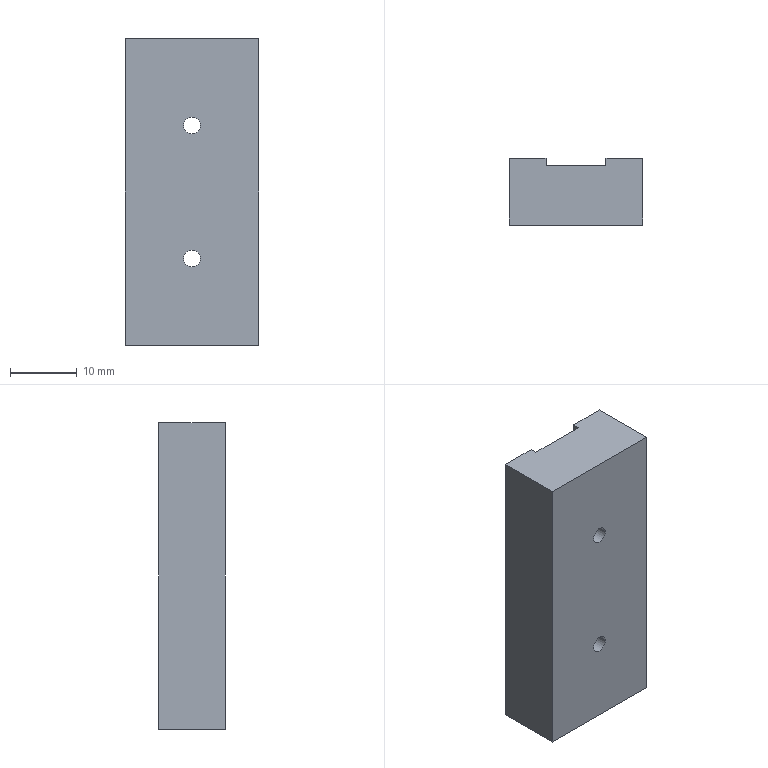Component | SolidWorks | P-SLJ-004-3_P-SLJ-004-002-1 | 1 solid | 22 faces | box 20 x 10 x 46 mm | volume 8495 mm3 | plane 10 | cylinder 8 | cone 4 | commonest cylinder face diameters 3.3 x4 2.5 x4 | material A3
build123d program:
from build123d import *

# Parameters (mm, degrees)
EXTRUDE1_DEPTH        = 23
M3_TAPPED_HOLE1_D     = 2.5
M4_TAPPED_HOLE2_D     = 3.3
M4_TAPPED_HOLE2_DEPTH = 11.5
M4_TAPPED_HOLE2_TIP   = 0.9914


with BuildPart() as part:
    # Sketch2 → Extrude1 (new, symmetric)
    with BuildSketch(Plane(origin=(0, 0, 0), x_dir=(0, 0, -1), z_dir=(1, 0, 0))):
        Polygon((4.5, 5), (10, 5), (10, -5), (-10, -5), (-10, 5), (-4.5, 5), (-4.5, 4), (4.5, 4), align=None)
    extrude(amount=EXTRUDE1_DEPTH, both=True)

    # M3 Tapped Hole1 (through all)
    with Locations(Plane(origin=(0, 4, 0), x_dir=(1, 0, 0), z_dir=(0, 1, 0))):
        with Locations((-10, 0), (10, 0)):
            Hole(M3_TAPPED_HOLE1_D / 2)

    # M4 Tapped Hole2
    with Locations(Plane.ZY.offset(23)):
        with Locations((5, 0), (-5, 0)):
            Hole(M4_TAPPED_HOLE2_D / 2, depth=M4_TAPPED_HOLE2_DEPTH)
            with Locations((0, 0, -(M4_TAPPED_HOLE2_DEPTH + M4_TAPPED_HOLE2_TIP / 2))):  # 118° drill point
                Cone(0, M4_TAPPED_HOLE2_D / 2, M4_TAPPED_HOLE2_TIP, mode=Mode.SUBTRACT)


solid = part.part

# Placed as in the assembly
solid = solid.moved(Location((-201.5, -45, 1287.634), (0, -90, 0)))
STEP:
#1=CARTESIAN_POINT('',(-8.065,-1.772,50.241));
#2=VERTEX_POINT('',#1);
#3=CARTESIAN_POINT('',(-8.195,-1.772,50.241));
#4=VERTEX_POINT('',#3);
#5=CARTESIAN_POINT('',(-8.13,-1.772,50.241));
#6=DIRECTION('',(-0.,0.,-1.));
#7=DIRECTION('',(-1.,0.,0.));
#8=AXIS2_PLACEMENT_3D('',#5,#6,#7);
#9=CIRCLE('',#8,0.06496);
#10=EDGE_CURVE('',#2,#4,#9,.T.);
#11=ORIENTED_EDGE('',*,*,#10,.F.);
#12=CARTESIAN_POINT('',(-8.065,-1.772,49.789));
#13=VERTEX_POINT('',#12);
#14=CARTESIAN_POINT('',(-8.065,-1.772,49.789));
#15=DIRECTION('',(-0.,0.,-1.));
#16=VECTOR('',#15,39.37);
#17=LINE('',#14,#16);
#18=EDGE_CURVE('',#2,#13,#17,.T.);
#19=ORIENTED_EDGE('',*,*,#18,.T.);
#20=CARTESIAN_POINT('',(-8.195,-1.772,49.789));
#21=VERTEX_POINT('',#20);
#22=CARTESIAN_POINT('',(-8.13,-1.772,49.789));
#23=DIRECTION('',(-0.,0.,-1.));
#24=DIRECTION('',(-1.,0.,0.));
#25=AXIS2_PLACEMENT_3D('',#22,#23,#24);
#26=CIRCLE('',#25,0.06496);
#27=EDGE_CURVE('',#13,#21,#26,.T.);
#28=ORIENTED_EDGE('',*,*,#27,.T.);
#29=CARTESIAN_POINT('',(-8.195,-1.772,49.789));
#30=DIRECTION('',(-0.,0.,-1.));
#31=VECTOR('',#30,39.37);
#32=LINE('',#29,#31);
#33=EDGE_CURVE('',#4,#21,#32,.T.);
#34=ORIENTED_EDGE('',*,*,#33,.F.);
#35=EDGE_LOOP('',(#11,#19,#28,#34));
#36=FACE_OUTER_BOUND('',#35,.T.);
#37=CARTESIAN_POINT('',(-8.13,-1.772,49.789));
#38=DIRECTION('',(-0.,0.,-1.));
#39=DIRECTION('',(-1.,0.,0.));
#40=AXIS2_PLACEMENT_3D('',#37,#38,#39);
#41=CYLINDRICAL_SURFACE('',#40,0.06496);
#42=ADVANCED_FACE('',(#36),#41,.F.);
#43=CARTESIAN_POINT('',(-8.13,-1.772,50.281));
#44=VERTEX_POINT('',#43);
#45=CARTESIAN_POINT('',(-8.195,-1.772,50.241));
#46=DIRECTION('',(-0.8572,0.,-0.515));
#47=VECTOR('',#46,39.37);
#48=LINE('',#45,#47);
#49=EDGE_CURVE('',#44,#4,#48,.T.);
#50=ORIENTED_EDGE('',*,*,#49,.F.);
#51=CARTESIAN_POINT('',(-8.065,-1.772,50.241));
#52=DIRECTION('',(0.8572,0.,-0.515));
#53=VECTOR('',#52,39.37);
#54=LINE('',#51,#53);
#55=EDGE_CURVE('',#44,#2,#54,.T.);
#56=ORIENTED_EDGE('',*,*,#55,.T.);
#57=ORIENTED_EDGE('',*,*,#10,.T.);
#58=EDGE_LOOP('',(#50,#56,#57));
#59=FACE_OUTER_BOUND('',#58,.T.);
#60=CARTESIAN_POINT('',(-8.13,-1.772,50.241));
#61=DIRECTION('',(-0.,0.,-1.));
#62=DIRECTION('',(-1.,0.,0.));
#63=AXIS2_PLACEMENT_3D('',#60,#61,#62);
#64=CONICAL_SURFACE('',#63,0.06496,1.03);
#65=ADVANCED_FACE('',(#59),#64,.F.);
#66=CARTESIAN_POINT('',(-7.671,-1.772,50.241));
#67=VERTEX_POINT('',#66);
#68=CARTESIAN_POINT('',(-7.801,-1.772,50.241));
#69=VERTEX_POINT('',#68);
#70=CARTESIAN_POINT('',(-7.736,-1.772,50.241));
#71=DIRECTION('',(-0.,0.,-1.));
#72=DIRECTION('',(-1.,0.,0.));
#73=AXIS2_PLACEMENT_3D('',#70,#71,#72);
#74=CIRCLE('',#73,0.06496);
#75=EDGE_CURVE('',#67,#69,#74,.T.);
#76=ORIENTED_EDGE('',*,*,#75,.F.);
#77=CARTESIAN_POINT('',(-7.671,-1.772,49.789));
#78=VERTEX_POINT('',#77);
#79=CARTESIAN_POINT('',(-7.671,-1.772,49.789));
#80=DIRECTION('',(-0.,0.,-1.));
#81=VECTOR('',#80,39.37);
#82=LINE('',#79,#81);
#83=EDGE_CURVE('',#67,#78,#82,.T.);
#84=ORIENTED_EDGE('',*,*,#83,.T.);
#85=CARTESIAN_POINT('',(-7.801,-1.772,49.789));
#86=VERTEX_POINT('',#85);
#87=CARTESIAN_POINT('',(-7.736,-1.772,49.789));
#88=DIRECTION('',(-0.,0.,-1.));
#89=DIRECTION('',(-1.,0.,0.));
#90=AXIS2_PLACEMENT_3D('',#87,#88,#89);
#91=CIRCLE('',#90,0.06496);
#92=EDGE_CURVE('',#78,#86,#91,.T.);
#93=ORIENTED_EDGE('',*,*,#92,.T.);
#94=CARTESIAN_POINT('',(-7.801,-1.772,49.789));
#95=DIRECTION('',(-0.,0.,-1.));
#96=VECTOR('',#95,39.37);
#97=LINE('',#94,#96);
#98=EDGE_CURVE('',#69,#86,#97,.T.);
#99=ORIENTED_EDGE('',*,*,#98,.F.);
#100=EDGE_LOOP('',(#76,#84,#93,#99));
#101=FACE_OUTER_BOUND('',#100,.T.);
#102=CARTESIAN_POINT('',(-7.736,-1.772,49.789));
#103=DIRECTION('',(-0.,0.,-1.));
#104=DIRECTION('',(-1.,0.,0.));
#105=AXIS2_PLACEMENT_3D('',#102,#103,#104);
#106=CYLINDRICAL_SURFACE('',#105,0.06496);
#107=ADVANCED_FACE('',(#101),#106,.F.);
#108=CARTESIAN_POINT('',(-7.736,-1.772,50.281));
#109=VERTEX_POINT('',#108);
#110=CARTESIAN_POINT('',(-7.801,-1.772,50.241));
#111=DIRECTION('',(-0.8572,0.,-0.515));
#112=VECTOR('',#111,39.37);
#113=LINE('',#110,#112);
#114=EDGE_CURVE('',#109,#69,#113,.T.);
#115=ORIENTED_EDGE('',*,*,#114,.F.);
#116=CARTESIAN_POINT('',(-7.671,-1.772,50.241));
#117=DIRECTION('',(0.8572,0.,-0.515));
#118=VECTOR('',#117,39.37);
#119=LINE('',#116,#118);
#120=EDGE_CURVE('',#109,#67,#119,.T.);
#121=ORIENTED_EDGE('',*,*,#120,.T.);
#122=ORIENTED_EDGE('',*,*,#75,.T.);
#123=EDGE_LOOP('',(#115,#121,#122));
#124=FACE_OUTER_BOUND('',#123,.T.);
#125=CARTESIAN_POINT('',(-7.736,-1.772,50.241));
#126=DIRECTION('',(-0.,0.,-1.));
#127=DIRECTION('',(-1.,0.,0.));
#128=AXIS2_PLACEMENT_3D('',#125,#126,#127);
#129=CONICAL_SURFACE('',#128,0.06496,1.03);
#130=ADVANCED_FACE('',(#124),#129,.F.);
#131=CARTESIAN_POINT('',(-7.884,-1.969,50.301));
#132=VERTEX_POINT('',#131);
#133=CARTESIAN_POINT('',(-7.982,-1.969,50.301));
#134=VERTEX_POINT('',#133);
#135=CARTESIAN_POINT('',(-7.933,-1.969,50.301));
#136=DIRECTION('',(0.,1.,0.));
#137=DIRECTION('',(-1.,0.,0.));
#138=AXIS2_PLACEMENT_3D('',#135,#136,#137);
#139=CIRCLE('',#138,0.04921);
#140=EDGE_CURVE('',#132,#134,#139,.T.);
#141=ORIENTED_EDGE('',*,*,#140,.F.);
#142=CARTESIAN_POINT('',(-7.884,-1.614,50.301));
#143=VERTEX_POINT('',#142);
#144=CARTESIAN_POINT('',(-7.884,-1.614,50.301));
#145=DIRECTION('',(0.,1.,0.));
#146=VECTOR('',#145,39.37);
#147=LINE('',#144,#146);
#148=EDGE_CURVE('',#132,#143,#147,.T.);
#149=ORIENTED_EDGE('',*,*,#148,.T.);
#150=CARTESIAN_POINT('',(-7.982,-1.614,50.301));
#151=VERTEX_POINT('',#150);
#152=CARTESIAN_POINT('',(-7.933,-1.614,50.301));
#153=DIRECTION('',(0.,1.,0.));
#154=DIRECTION('',(-1.,0.,0.));
#155=AXIS2_PLACEMENT_3D('',#152,#153,#154);
#156=CIRCLE('',#155,0.04921);
#157=EDGE_CURVE('',#143,#151,#156,.T.);
#158=ORIENTED_EDGE('',*,*,#157,.T.);
#159=CARTESIAN_POINT('',(-7.982,-1.614,50.301));
#160=DIRECTION('',(0.,1.,0.));
#161=VECTOR('',#160,39.37);
#162=LINE('',#159,#161);
#163=EDGE_CURVE('',#134,#151,#162,.T.);
#164=ORIENTED_EDGE('',*,*,#163,.F.);
#165=EDGE_LOOP('',(#141,#149,#158,#164));
#166=FACE_OUTER_BOUND('',#165,.T.);
#167=CARTESIAN_POINT('',(-7.933,-1.614,50.301));
#168=DIRECTION('',(0.,1.,0.));
#169=DIRECTION('',(-1.,0.,0.));
#170=AXIS2_PLACEMENT_3D('',#167,#168,#169);
#171=CYLINDRICAL_SURFACE('',#170,0.04921);
#172=ADVANCED_FACE('',(#166),#171,.F.);
#173=CARTESIAN_POINT('',(-7.884,-1.969,51.088));
#174=VERTEX_POINT('',#173);
#175=CARTESIAN_POINT('',(-7.982,-1.969,51.088));
#176=VERTEX_POINT('',#175);
#177=CARTESIAN_POINT('',(-7.933,-1.969,51.088));
#178=DIRECTION('',(0.,1.,0.));
#179=DIRECTION('',(-1.,0.,0.));
#180=AXIS2_PLACEMENT_3D('',#177,#178,#179);
#181=CIRCLE('',#180,0.04921);
#182=EDGE_CURVE('',#174,#176,#181,.T.);
#183=ORIENTED_EDGE('',*,*,#182,.F.);
#184=CARTESIAN_POINT('',(-7.884,-1.614,51.088));
#185=VERTEX_POINT('',#184);
#186=CARTESIAN_POINT('',(-7.884,-1.614,51.088));
#187=DIRECTION('',(0.,1.,0.));
#188=VECTOR('',#187,39.37);
#189=LINE('',#186,#188);
#190=EDGE_CURVE('',#174,#185,#189,.T.);
#191=ORIENTED_EDGE('',*,*,#190,.T.);
#192=CARTESIAN_POINT('',(-7.982,-1.614,51.088));
#193=VERTEX_POINT('',#192);
#194=CARTESIAN_POINT('',(-7.933,-1.614,51.088));
#195=DIRECTION('',(0.,1.,0.));
#196=DIRECTION('',(-1.,0.,0.));
#197=AXIS2_PLACEMENT_3D('',#194,#195,#196);
#198=CIRCLE('',#197,0.04921);
#199=EDGE_CURVE('',#185,#193,#198,.T.);
#200=ORIENTED_EDGE('',*,*,#199,.T.);
#201=CARTESIAN_POINT('',(-7.982,-1.614,51.088));
#202=DIRECTION('',(0.,1.,0.));
#203=VECTOR('',#202,39.37);
#204=LINE('',#201,#203);
#205=EDGE_CURVE('',#176,#193,#204,.T.);
#206=ORIENTED_EDGE('',*,*,#205,.F.);
#207=EDGE_LOOP('',(#183,#191,#200,#206));
#208=FACE_OUTER_BOUND('',#207,.T.);
#209=CARTESIAN_POINT('',(-7.933,-1.614,51.088));
#210=DIRECTION('',(0.,1.,0.));
#211=DIRECTION('',(-1.,0.,0.));
#212=AXIS2_PLACEMENT_3D('',#209,#210,#211);
#213=CYLINDRICAL_SURFACE('',#212,0.04921);
#214=ADVANCED_FACE('',(#208),#213,.F.);
#215=CARTESIAN_POINT('',(-7.539,-1.969,49.789));
#216=VERTEX_POINT('',#215);
#217=CARTESIAN_POINT('',(-7.539,-1.575,49.789));
#218=VERTEX_POINT('',#217);
#219=CARTESIAN_POINT('',(-7.539,-1.969,49.789));
#220=DIRECTION('',(-0.,1.,0.));
#221=VECTOR('',#220,39.37);
#222=LINE('',#219,#221);
#223=EDGE_CURVE('',#216,#218,#222,.T.);
#224=ORIENTED_EDGE('',*,*,#223,.T.);
#225=CARTESIAN_POINT('',(-7.539,-1.575,51.6));
#226=VERTEX_POINT('',#225);
#227=CARTESIAN_POINT('',(-7.539,-1.575,51.6));
#228=DIRECTION('',(-0.,0.,-1.));
#229=VECTOR('',#228,39.37);
#230=LINE('',#227,#229);
#231=EDGE_CURVE('',#226,#218,#230,.T.);
#232=ORIENTED_EDGE('',*,*,#231,.F.);
#233=CARTESIAN_POINT('',(-7.539,-1.969,51.6));
#234=VERTEX_POINT('',#233);
#235=CARTESIAN_POINT('',(-7.539,-1.969,51.6));
#236=DIRECTION('',(-0.,1.,0.));
#237=VECTOR('',#236,39.37);
#238=LINE('',#235,#237);
#239=EDGE_CURVE('',#234,#226,#238,.T.);
#240=ORIENTED_EDGE('',*,*,#239,.F.);
#241=CARTESIAN_POINT('',(-7.539,-1.969,51.6));
#242=DIRECTION('',(-0.,0.,-1.));
#243=VECTOR('',#242,39.37);
#244=LINE('',#241,#243);
#245=EDGE_CURVE('',#234,#216,#244,.T.);
#246=ORIENTED_EDGE('',*,*,#245,.T.);
#247=EDGE_LOOP('',(#224,#232,#240,#246));
#248=FACE_OUTER_BOUND('',#247,.T.);
#249=CARTESIAN_POINT('',(-7.539,-1.969,51.6));
#250=DIRECTION('',(-1.,-0.,0.));
#251=DIRECTION('',(0.,-1.,-0.));
#252=AXIS2_PLACEMENT_3D('',#249,#250,#251);
#253=PLANE('',#252);
#254=ADVANCED_FACE('',(#248),#253,.F.);
#255=CARTESIAN_POINT('',(-7.756,-1.575,49.789));
#256=VERTEX_POINT('',#255);
#257=CARTESIAN_POINT('',(-7.756,-1.575,49.789));
#258=DIRECTION('',(-1.,0.,0.));
#259=VECTOR('',#258,39.37);
#260=LINE('',#257,#259);
#261=EDGE_CURVE('',#218,#256,#260,.T.);
#262=ORIENTED_EDGE('',*,*,#261,.T.);
#263=CARTESIAN_POINT('',(-7.756,-1.575,51.6));
#264=VERTEX_POINT('',#263);
#265=CARTESIAN_POINT('',(-7.756,-1.575,51.6));
#266=DIRECTION('',(-0.,0.,-1.));
#267=VECTOR('',#266,39.37);
#268=LINE('',#265,#267);
#269=EDGE_CURVE('',#264,#256,#268,.T.);
#270=ORIENTED_EDGE('',*,*,#269,.F.);
#271=CARTESIAN_POINT('',(-7.756,-1.575,51.6));
#272=DIRECTION('',(-1.,0.,0.));
#273=VECTOR('',#272,39.37);
#274=LINE('',#271,#273);
#275=EDGE_CURVE('',#226,#264,#274,.T.);
#276=ORIENTED_EDGE('',*,*,#275,.F.);
#277=ORIENTED_EDGE('',*,*,#231,.T.);
#278=EDGE_LOOP('',(#262,#270,#276,#277));
#279=FACE_OUTER_BOUND('',#278,.T.);
#280=CARTESIAN_POINT('',(-7.756,-1.575,51.6));
#281=DIRECTION('',(-0.,-1.,-0.));
#282=DIRECTION('',(1.,-0.,-0.));
#283=AXIS2_PLACEMENT_3D('',#280,#281,#282);
#284=PLANE('',#283);
#285=ADVANCED_FACE('',(#279),#284,.F.);
#286=CARTESIAN_POINT('',(-7.756,-1.614,49.789));
#287=VERTEX_POINT('',#286);
#288=CARTESIAN_POINT('',(-7.756,-1.575,49.789));
#289=DIRECTION('',(-0.,-1.,-0.));
#290=VECTOR('',#289,39.37);
#291=LINE('',#288,#290);
#292=EDGE_CURVE('',#256,#287,#291,.T.);
#293=ORIENTED_EDGE('',*,*,#292,.T.);
#294=CARTESIAN_POINT('',(-7.756,-1.614,51.6));
#295=VERTEX_POINT('',#294);
#296=CARTESIAN_POINT('',(-7.756,-1.614,51.6));
#297=DIRECTION('',(-0.,0.,-1.));
#298=VECTOR('',#297,39.37);
#299=LINE('',#296,#298);
#300=EDGE_CURVE('',#295,#287,#299,.T.);
#301=ORIENTED_EDGE('',*,*,#300,.F.);
#302=CARTESIAN_POINT('',(-7.756,-1.575,51.6));
#303=DIRECTION('',(-0.,-1.,-0.));
#304=VECTOR('',#303,39.37);
#305=LINE('',#302,#304);
#306=EDGE_CURVE('',#264,#295,#305,.T.);
#307=ORIENTED_EDGE('',*,*,#306,.F.);
#308=ORIENTED_EDGE('',*,*,#269,.T.);
#309=EDGE_LOOP('',(#293,#301,#307,#308));
#310=FACE_OUTER_BOUND('',#309,.T.);
#311=CARTESIAN_POINT('',(-7.756,-1.575,51.6));
#312=DIRECTION('',(1.,-0.,-0.));
#313=DIRECTION('',(-0.,0.,-1.));
#314=AXIS2_PLACEMENT_3D('',#311,#312,#313);
#315=PLANE('',#314);
#316=ADVANCED_FACE('',(#310),#315,.F.);
#317=CARTESIAN_POINT('',(-7.933,-1.614,50.301));
#318=DIRECTION('',(0.,1.,0.));
#319=DIRECTION('',(-1.,0.,0.));
#320=AXIS2_PLACEMENT_3D('',#317,#318,#319);
#321=CIRCLE('',#320,0.04921);
#322=EDGE_CURVE('',#151,#143,#321,.T.);
#323=ORIENTED_EDGE('',*,*,#322,.F.);
#324=ORIENTED_EDGE('',*,*,#157,.F.);
#325=EDGE_LOOP('',(#323,#324));
#326=FACE_BOUND('',#325,.T.);
#327=CARTESIAN_POINT('',(-7.933,-1.614,51.088));
#328=DIRECTION('',(0.,1.,0.));
#329=DIRECTION('',(-1.,0.,0.));
#330=AXIS2_PLACEMENT_3D('',#327,#328,#329);
#331=CIRCLE('',#330,0.04921);
#332=EDGE_CURVE('',#193,#185,#331,.T.);
#333=ORIENTED_EDGE('',*,*,#332,.F.);
#334=ORIENTED_EDGE('',*,*,#199,.F.);
#335=EDGE_LOOP('',(#333,#334));
#336=FACE_BOUND('',#335,.T.);
#337=CARTESIAN_POINT('',(-8.11,-1.614,49.789));
#338=VERTEX_POINT('',#337);
#339=CARTESIAN_POINT('',(-8.11,-1.614,49.789));
#340=DIRECTION('',(-1.,0.,0.));
#341=VECTOR('',#340,39.37);
#342=LINE('',#339,#341);
#343=EDGE_CURVE('',#287,#338,#342,.T.);
#344=ORIENTED_EDGE('',*,*,#343,.T.);
#345=CARTESIAN_POINT('',(-8.11,-1.614,51.6));
#346=VERTEX_POINT('',#345);
#347=CARTESIAN_POINT('',(-8.11,-1.614,51.6));
#348=DIRECTION('',(-0.,0.,-1.));
#349=VECTOR('',#348,39.37);
#350=LINE('',#347,#349);
#351=EDGE_CURVE('',#346,#338,#350,.T.);
#352=ORIENTED_EDGE('',*,*,#351,.F.);
#353=CARTESIAN_POINT('',(-8.11,-1.614,51.6));
#354=DIRECTION('',(-1.,0.,0.));
#355=VECTOR('',#354,39.37);
#356=LINE('',#353,#355);
#357=EDGE_CURVE('',#295,#346,#356,.T.);
#358=ORIENTED_EDGE('',*,*,#357,.F.);
#359=ORIENTED_EDGE('',*,*,#300,.T.);
#360=EDGE_LOOP('',(#344,#352,#358,#359));
#361=FACE_OUTER_BOUND('',#360,.T.);
#362=CARTESIAN_POINT('',(-8.11,-1.614,51.6));
#363=DIRECTION('',(-0.,-1.,-0.));
#364=DIRECTION('',(1.,-0.,-0.));
#365=AXIS2_PLACEMENT_3D('',#362,#363,#364);
#366=PLANE('',#365);
#367=ADVANCED_FACE('',(#326,#336,#361),#366,.F.);
#368=CARTESIAN_POINT('',(-8.11,-1.575,49.789));
#369=VERTEX_POINT('',#368);
#370=CARTESIAN_POINT('',(-8.11,-1.575,49.789));
#371=DIRECTION('',(0.,1.,0.));
#372=VECTOR('',#371,39.37);
#373=LINE('',#370,#372);
#374=EDGE_CURVE('',#338,#369,#373,.T.);
#375=ORIENTED_EDGE('',*,*,#374,.T.);
#376=CARTESIAN_POINT('',(-8.11,-1.575,51.6));
#377=VERTEX_POINT('',#376);
#378=CARTESIAN_POINT('',(-8.11,-1.575,51.6));
#379=DIRECTION('',(-0.,0.,-1.));
#380=VECTOR('',#379,39.37);
#381=LINE('',#378,#380);
#382=EDGE_CURVE('',#377,#369,#381,.T.);
#383=ORIENTED_EDGE('',*,*,#382,.F.);
#384=CARTESIAN_POINT('',(-8.11,-1.575,51.6));
#385=DIRECTION('',(0.,1.,0.));
#386=VECTOR('',#385,39.37);
#387=LINE('',#384,#386);
#388=EDGE_CURVE('',#346,#377,#387,.T.);
#389=ORIENTED_EDGE('',*,*,#388,.F.);
#390=ORIENTED_EDGE('',*,*,#351,.T.);
#391=EDGE_LOOP('',(#375,#383,#389,#390));
#392=FACE_OUTER_BOUND('',#391,.T.);
#393=CARTESIAN_POINT('',(-8.11,-1.575,51.6));
#394=DIRECTION('',(-1.,0.,0.));
#395=DIRECTION('',(0.,-0.,1.));
#396=AXIS2_PLACEMENT_3D('',#393,#394,#395);
#397=PLANE('',#396);
#398=ADVANCED_FACE('',(#392),#397,.F.);
#399=CARTESIAN_POINT('',(-8.327,-1.575,49.789));
#400=VERTEX_POINT('',#399);
#401=CARTESIAN_POINT('',(-8.327,-1.575,49.789));
#402=DIRECTION('',(-1.,-0.,0.));
#403=VECTOR('',#402,39.37);
#404=LINE('',#401,#403);
#405=EDGE_CURVE('',#369,#400,#404,.T.);
#406=ORIENTED_EDGE('',*,*,#405,.T.);
#407=CARTESIAN_POINT('',(-8.327,-1.575,51.6));
#408=VERTEX_POINT('',#407);
#409=CARTESIAN_POINT('',(-8.327,-1.575,51.6));
#410=DIRECTION('',(-0.,0.,-1.));
#411=VECTOR('',#410,39.37);
#412=LINE('',#409,#411);
#413=EDGE_CURVE('',#408,#400,#412,.T.);
#414=ORIENTED_EDGE('',*,*,#413,.F.);
#415=CARTESIAN_POINT('',(-8.327,-1.575,51.6));
#416=DIRECTION('',(-1.,-0.,0.));
#417=VECTOR('',#416,39.37);
#418=LINE('',#415,#417);
#419=EDGE_CURVE('',#377,#408,#418,.T.);
#420=ORIENTED_EDGE('',*,*,#419,.F.);
#421=ORIENTED_EDGE('',*,*,#382,.T.);
#422=EDGE_LOOP('',(#406,#414,#420,#421));
#423=FACE_OUTER_BOUND('',#422,.T.);
#424=CARTESIAN_POINT('',(-8.327,-1.575,51.6));
#425=DIRECTION('',(0.,-1.,-0.));
#426=DIRECTION('',(1.,0.,-0.));
#427=AXIS2_PLACEMENT_3D('',#424,#425,#426);
#428=PLANE('',#427);
#429=ADVANCED_FACE('',(#423),#428,.F.);
#430=CARTESIAN_POINT('',(-8.327,-1.969,49.789));
#431=VERTEX_POINT('',#430);
#432=CARTESIAN_POINT('',(-8.327,-1.969,49.789));
#433=DIRECTION('',(-0.,-1.,-0.));
#434=VECTOR('',#433,39.37);
#435=LINE('',#432,#434);
#436=EDGE_CURVE('',#400,#431,#435,.T.);
#437=ORIENTED_EDGE('',*,*,#436,.T.);
#438=CARTESIAN_POINT('',(-8.327,-1.969,51.6));
#439=VERTEX_POINT('',#438);
#440=CARTESIAN_POINT('',(-8.327,-1.969,51.6));
#441=DIRECTION('',(-0.,0.,-1.));
#442=VECTOR('',#441,39.37);
#443=LINE('',#440,#442);
#444=EDGE_CURVE('',#439,#431,#443,.T.);
#445=ORIENTED_EDGE('',*,*,#444,.F.);
#446=CARTESIAN_POINT('',(-8.327,-1.969,51.6));
#447=DIRECTION('',(-0.,-1.,-0.));
#448=VECTOR('',#447,39.37);
#449=LINE('',#446,#448);
#450=EDGE_CURVE('',#408,#439,#449,.T.);
#451=ORIENTED_EDGE('',*,*,#450,.F.);
#452=ORIENTED_EDGE('',*,*,#413,.T.);
#453=EDGE_LOOP('',(#437,#445,#451,#452));
#454=FACE_OUTER_BOUND('',#453,.T.);
#455=CARTESIAN_POINT('',(-8.327,-1.969,51.6));
#456=DIRECTION('',(1.,-0.,-0.));
#457=DIRECTION('',(-0.,0.,-1.));
#458=AXIS2_PLACEMENT_3D('',#455,#456,#457);
#459=PLANE('',#458);
#460=ADVANCED_FACE('',(#454),#459,.F.);
#461=CARTESIAN_POINT('',(-7.933,-1.969,50.301));
#462=DIRECTION('',(0.,1.,0.));
#463=DIRECTION('',(-1.,0.,0.));
#464=AXIS2_PLACEMENT_3D('',#461,#462,#463);
#465=CIRCLE('',#464,0.04921);
#466=EDGE_CURVE('',#134,#132,#465,.T.);
#467=ORIENTED_EDGE('',*,*,#466,.T.);
#468=ORIENTED_EDGE('',*,*,#140,.T.);
#469=EDGE_LOOP('',(#467,#468));
#470=FACE_BOUND('',#469,.T.);
#471=CARTESIAN_POINT('',(-7.933,-1.969,51.088));
#472=DIRECTION('',(0.,1.,0.));
#473=DIRECTION('',(-1.,0.,0.));
#474=AXIS2_PLACEMENT_3D('',#471,#472,#473);
#475=CIRCLE('',#474,0.04921);
#476=EDGE_CURVE('',#176,#174,#475,.T.);
#477=ORIENTED_EDGE('',*,*,#476,.T.);
#478=ORIENTED_EDGE('',*,*,#182,.T.);
#479=EDGE_LOOP('',(#477,#478));
#480=FACE_BOUND('',#479,.T.);
#481=CARTESIAN_POINT('',(-8.327,-1.969,49.789));
#482=DIRECTION('',(1.,-0.,-0.));
#483=VECTOR('',#482,39.37);
#484=LINE('',#481,#483);
#485=EDGE_CURVE('',#431,#216,#484,.T.);
#486=ORIENTED_EDGE('',*,*,#485,.T.);
#487=ORIENTED_EDGE('',*,*,#245,.F.);
#488=CARTESIAN_POINT('',(-8.327,-1.969,51.6));
#489=DIRECTION('',(1.,-0.,-0.));
#490=VECTOR('',#489,39.37);
#491=LINE('',#488,#490);
#492=EDGE_CURVE('',#439,#234,#491,.T.);
#493=ORIENTED_EDGE('',*,*,#492,.F.);
#494=ORIENTED_EDGE('',*,*,#444,.T.);
#495=EDGE_LOOP('',(#486,#487,#493,#494));
#496=FACE_OUTER_BOUND('',#495,.T.);
#497=CARTESIAN_POINT('',(-8.327,-1.969,51.6));
#498=DIRECTION('',(0.,1.,0.));
#499=DIRECTION('',(-1.,0.,0.));
#500=AXIS2_PLACEMENT_3D('',#497,#498,#499);
#501=PLANE('',#500);
#502=ADVANCED_FACE('',(#470,#480,#496),#501,.F.);
#503=ORIENTED_EDGE('',*,*,#239,.T.);
#504=ORIENTED_EDGE('',*,*,#275,.T.);
#505=ORIENTED_EDGE('',*,*,#306,.T.);
#506=ORIENTED_EDGE('',*,*,#357,.T.);
#507=ORIENTED_EDGE('',*,*,#388,.T.);
#508=ORIENTED_EDGE('',*,*,#419,.T.);
#509=ORIENTED_EDGE('',*,*,#450,.T.);
#510=ORIENTED_EDGE('',*,*,#492,.T.);
#511=EDGE_LOOP('',(#503,#504,#505,#506,#507,#508,#509,#510));
#512=FACE_OUTER_BOUND('',#511,.T.);
#513=CARTESIAN_POINT('',(-7.933,-1.772,51.6));
#514=DIRECTION('',(-0.,0.,-1.));
#515=DIRECTION('',(-1.,0.,0.));
#516=AXIS2_PLACEMENT_3D('',#513,#514,#515);
#517=PLANE('',#516);
#518=ADVANCED_FACE('',(#512),#517,.F.);
#519=CARTESIAN_POINT('',(-8.13,-1.772,49.789));
#520=DIRECTION('',(-0.,0.,-1.));
#521=DIRECTION('',(-1.,0.,0.));
#522=AXIS2_PLACEMENT_3D('',#519,#520,#521);
#523=CIRCLE('',#522,0.06496);
#524=EDGE_CURVE('',#21,#13,#523,.T.);
#525=ORIENTED_EDGE('',*,*,#524,.F.);
#526=ORIENTED_EDGE('',*,*,#27,.F.);
#527=EDGE_LOOP('',(#525,#526));
#528=FACE_BOUND('',#527,.T.);
#529=CARTESIAN_POINT('',(-7.736,-1.772,49.789));
#530=DIRECTION('',(-0.,0.,-1.));
#531=DIRECTION('',(-1.,0.,0.));
#532=AXIS2_PLACEMENT_3D('',#529,#530,#531);
#533=CIRCLE('',#532,0.06496);
#534=EDGE_CURVE('',#86,#78,#533,.T.);
#535=ORIENTED_EDGE('',*,*,#534,.F.);
#536=ORIENTED_EDGE('',*,*,#92,.F.);
#537=EDGE_LOOP('',(#535,#536));
#538=FACE_BOUND('',#537,.T.);
#539=ORIENTED_EDGE('',*,*,#223,.F.);
#540=ORIENTED_EDGE('',*,*,#485,.F.);
#541=ORIENTED_EDGE('',*,*,#436,.F.);
#542=ORIENTED_EDGE('',*,*,#405,.F.);
#543=ORIENTED_EDGE('',*,*,#374,.F.);
#544=ORIENTED_EDGE('',*,*,#343,.F.);
#545=ORIENTED_EDGE('',*,*,#292,.F.);
#546=ORIENTED_EDGE('',*,*,#261,.F.);
#547=EDGE_LOOP('',(#539,#540,#541,#542,#543,#544,#545,#546));
#548=FACE_OUTER_BOUND('',#547,.T.);
#549=CARTESIAN_POINT('',(-7.933,-1.772,49.789));
#550=DIRECTION('',(-0.,0.,-1.));
#551=DIRECTION('',(-1.,0.,0.));
#552=AXIS2_PLACEMENT_3D('',#549,#550,#551);
#553=PLANE('',#552);
#554=ADVANCED_FACE('',(#528,#538,#548),#553,.T.);
#555=ORIENTED_EDGE('',*,*,#190,.F.);
#556=ORIENTED_EDGE('',*,*,#476,.F.);
#557=ORIENTED_EDGE('',*,*,#205,.T.);
#558=ORIENTED_EDGE('',*,*,#332,.T.);
#559=EDGE_LOOP('',(#555,#556,#557,#558));
#560=FACE_OUTER_BOUND('',#559,.T.);
#561=CARTESIAN_POINT('',(-7.933,-1.614,51.088));
#562=DIRECTION('',(0.,1.,0.));
#563=DIRECTION('',(-1.,0.,0.));
#564=AXIS2_PLACEMENT_3D('',#561,#562,#563);
#565=CYLINDRICAL_SURFACE('',#564,0.04921);
#566=ADVANCED_FACE('',(#560),#565,.F.);
#567=ORIENTED_EDGE('',*,*,#148,.F.);
#568=ORIENTED_EDGE('',*,*,#466,.F.);
#569=ORIENTED_EDGE('',*,*,#163,.T.);
#570=ORIENTED_EDGE('',*,*,#322,.T.);
#571=EDGE_LOOP('',(#567,#568,#569,#570));
#572=FACE_OUTER_BOUND('',#571,.T.);
#573=CARTESIAN_POINT('',(-7.933,-1.614,50.301));
#574=DIRECTION('',(0.,1.,0.));
#575=DIRECTION('',(-1.,0.,0.));
#576=AXIS2_PLACEMENT_3D('',#573,#574,#575);
#577=CYLINDRICAL_SURFACE('',#576,0.04921);
#578=ADVANCED_FACE('',(#572),#577,.F.);
#579=ORIENTED_EDGE('',*,*,#120,.F.);
#580=ORIENTED_EDGE('',*,*,#114,.T.);
#581=CARTESIAN_POINT('',(-7.736,-1.772,50.241));
#582=DIRECTION('',(-0.,0.,-1.));
#583=DIRECTION('',(-1.,0.,0.));
#584=AXIS2_PLACEMENT_3D('',#581,#582,#583);
#585=CIRCLE('',#584,0.06496);
#586=EDGE_CURVE('',#69,#67,#585,.T.);
#587=ORIENTED_EDGE('',*,*,#586,.T.);
#588=EDGE_LOOP('',(#579,#580,#587));
#589=FACE_OUTER_BOUND('',#588,.T.);
#590=CARTESIAN_POINT('',(-7.736,-1.772,50.241));
#591=DIRECTION('',(-0.,0.,-1.));
#592=DIRECTION('',(-1.,0.,0.));
#593=AXIS2_PLACEMENT_3D('',#590,#591,#592);
#594=CONICAL_SURFACE('',#593,0.06496,1.03);
#595=ADVANCED_FACE('',(#589),#594,.F.);
#596=ORIENTED_EDGE('',*,*,#83,.F.);
#597=ORIENTED_EDGE('',*,*,#586,.F.);
#598=ORIENTED_EDGE('',*,*,#98,.T.);
#599=ORIENTED_EDGE('',*,*,#534,.T.);
#600=EDGE_LOOP('',(#596,#597,#598,#599));
#601=FACE_OUTER_BOUND('',#600,.T.);
#602=CARTESIAN_POINT('',(-7.736,-1.772,49.789));
#603=DIRECTION('',(-0.,0.,-1.));
#604=DIRECTION('',(-1.,0.,0.));
#605=AXIS2_PLACEMENT_3D('',#602,#603,#604);
#606=CYLINDRICAL_SURFACE('',#605,0.06496);
#607=ADVANCED_FACE('',(#601),#606,.F.);
#608=ORIENTED_EDGE('',*,*,#55,.F.);
#609=ORIENTED_EDGE('',*,*,#49,.T.);
#610=CARTESIAN_POINT('',(-8.13,-1.772,50.241));
#611=DIRECTION('',(-0.,0.,-1.));
#612=DIRECTION('',(-1.,0.,0.));
#613=AXIS2_PLACEMENT_3D('',#610,#611,#612);
#614=CIRCLE('',#613,0.06496);
#615=EDGE_CURVE('',#4,#2,#614,.T.);
#616=ORIENTED_EDGE('',*,*,#615,.T.);
#617=EDGE_LOOP('',(#608,#609,#616));
#618=FACE_OUTER_BOUND('',#617,.T.);
#619=CARTESIAN_POINT('',(-8.13,-1.772,50.241));
#620=DIRECTION('',(-0.,0.,-1.));
#621=DIRECTION('',(-1.,0.,0.));
#622=AXIS2_PLACEMENT_3D('',#619,#620,#621);
#623=CONICAL_SURFACE('',#622,0.06496,1.03);
#624=ADVANCED_FACE('',(#618),#623,.F.);
#625=ORIENTED_EDGE('',*,*,#18,.F.);
#626=ORIENTED_EDGE('',*,*,#615,.F.);
#627=ORIENTED_EDGE('',*,*,#33,.T.);
#628=ORIENTED_EDGE('',*,*,#524,.T.);
#629=EDGE_LOOP('',(#625,#626,#627,#628));
#630=FACE_OUTER_BOUND('',#629,.T.);
#631=CARTESIAN_POINT('',(-8.13,-1.772,49.789));
#632=DIRECTION('',(-0.,0.,-1.));
#633=DIRECTION('',(-1.,0.,0.));
#634=AXIS2_PLACEMENT_3D('',#631,#632,#633);
#635=CYLINDRICAL_SURFACE('',#634,0.06496);
#636=ADVANCED_FACE('',(#630),#635,.F.);
#637=CLOSED_SHELL('',(#42,#65,#107,#130,#172,#214,#254,#285,#316,#367,#398,#429,#460,#502,#518,#554,#566,#578,#595,#607,#624,#636));
#638=MANIFOLD_SOLID_BREP('',#637);
#639=CARTESIAN_POINT('',(0.,0.,0.));
#640=DIRECTION('',(0.,0.,1.));
#641=DIRECTION('',(1.,0.,0.));
#642=AXIS2_PLACEMENT_3D('',#639,#640,#641);
#643=(LENGTH_UNIT()NAMED_UNIT(*)SI_UNIT($,.METRE.));
#644=LENGTH_MEASURE_WITH_UNIT(LENGTH_MEASURE(0.0254),#643);
#645=DIMENSIONAL_EXPONENTS(1.,0.,0.,0.,0.,0.,0.);
#646=(CONVERSION_BASED_UNIT('',#644)LENGTH_UNIT()NAMED_UNIT(#645));
#647=UNCERTAINTY_MEASURE_WITH_UNIT(LENGTH_MEASURE(0.00001),#646,'','');
#648=(NAMED_UNIT(*)PLANE_ANGLE_UNIT()SI_UNIT($,.RADIAN.));
#649=(NAMED_UNIT(*)SI_UNIT($,.STERADIAN.)SOLID_ANGLE_UNIT());
#650=(GEOMETRIC_REPRESENTATION_CONTEXT(3)GLOBAL_UNCERTAINTY_ASSIGNED_CONTEXT((#647))GLOBAL_UNIT_ASSIGNED_CONTEXT((#646,#648,#649))REPRESENTATION_CONTEXT('',''));
#651=ADVANCED_BREP_SHAPE_REPRESENTATION('',(#638,#642),#650);
#652=COLOUR_RGB('',0.7922,0.8196,0.9333);
#653=FILL_AREA_STYLE_COLOUR('',#652);
#654=FILL_AREA_STYLE('',(#653));
#655=SURFACE_STYLE_FILL_AREA(#654);
#656=SURFACE_SIDE_STYLE('',(#655));
#657=SURFACE_STYLE_USAGE(.BOTH.,#656);
#658=PRESENTATION_STYLE_ASSIGNMENT((#657));
#659=STYLED_ITEM('',(#658),#638);
#660=PRESENTATION_LAYER_ASSIGNMENT('','',(#659));
#661=(LENGTH_UNIT()NAMED_UNIT(*)SI_UNIT($,.METRE.));
#662=LENGTH_MEASURE_WITH_UNIT(LENGTH_MEASURE(0.0254),#661);
#663=DIMENSIONAL_EXPONENTS(1.,0.,0.,0.,0.,0.,0.);
#664=(CONVERSION_BASED_UNIT('',#662)LENGTH_UNIT()NAMED_UNIT(#663));
#665=UNCERTAINTY_MEASURE_WITH_UNIT(LENGTH_MEASURE(0.00001),#664,'','');
#666=(NAMED_UNIT(*)PLANE_ANGLE_UNIT()SI_UNIT($,.RADIAN.));
#667=(NAMED_UNIT(*)SI_UNIT($,.STERADIAN.)SOLID_ANGLE_UNIT());
#668=(GEOMETRIC_REPRESENTATION_CONTEXT(3)GLOBAL_UNCERTAINTY_ASSIGNED_CONTEXT((#665))GLOBAL_UNIT_ASSIGNED_CONTEXT((#664,#666,#667))REPRESENTATION_CONTEXT('',''));
#669=MECHANICAL_DESIGN_GEOMETRIC_PRESENTATION_REPRESENTATION('',(#659),#668);